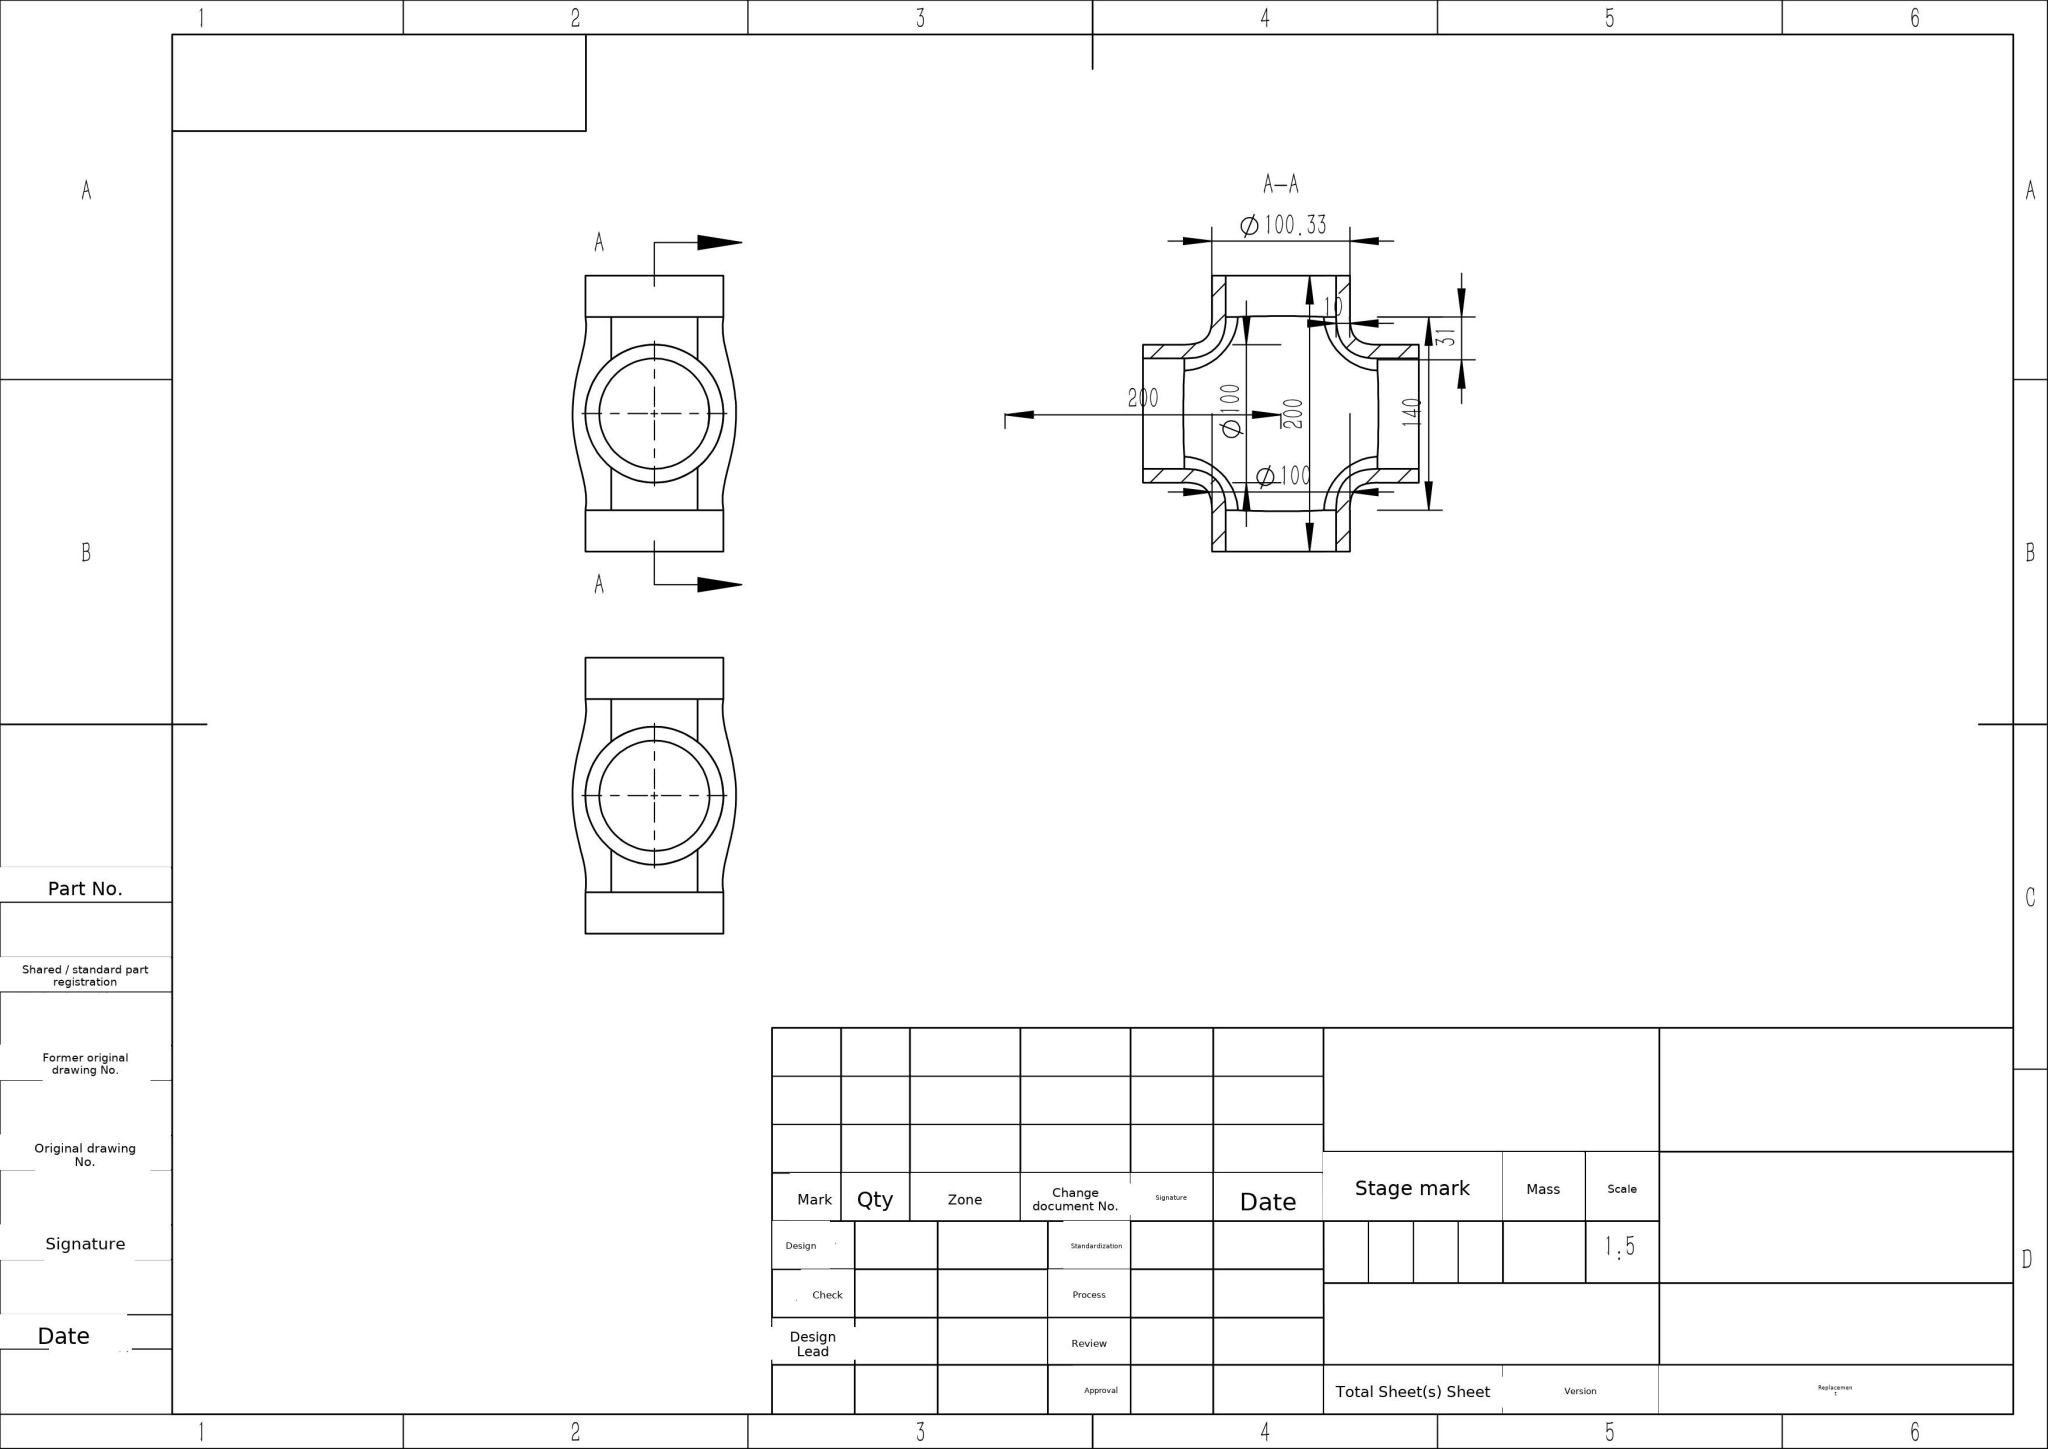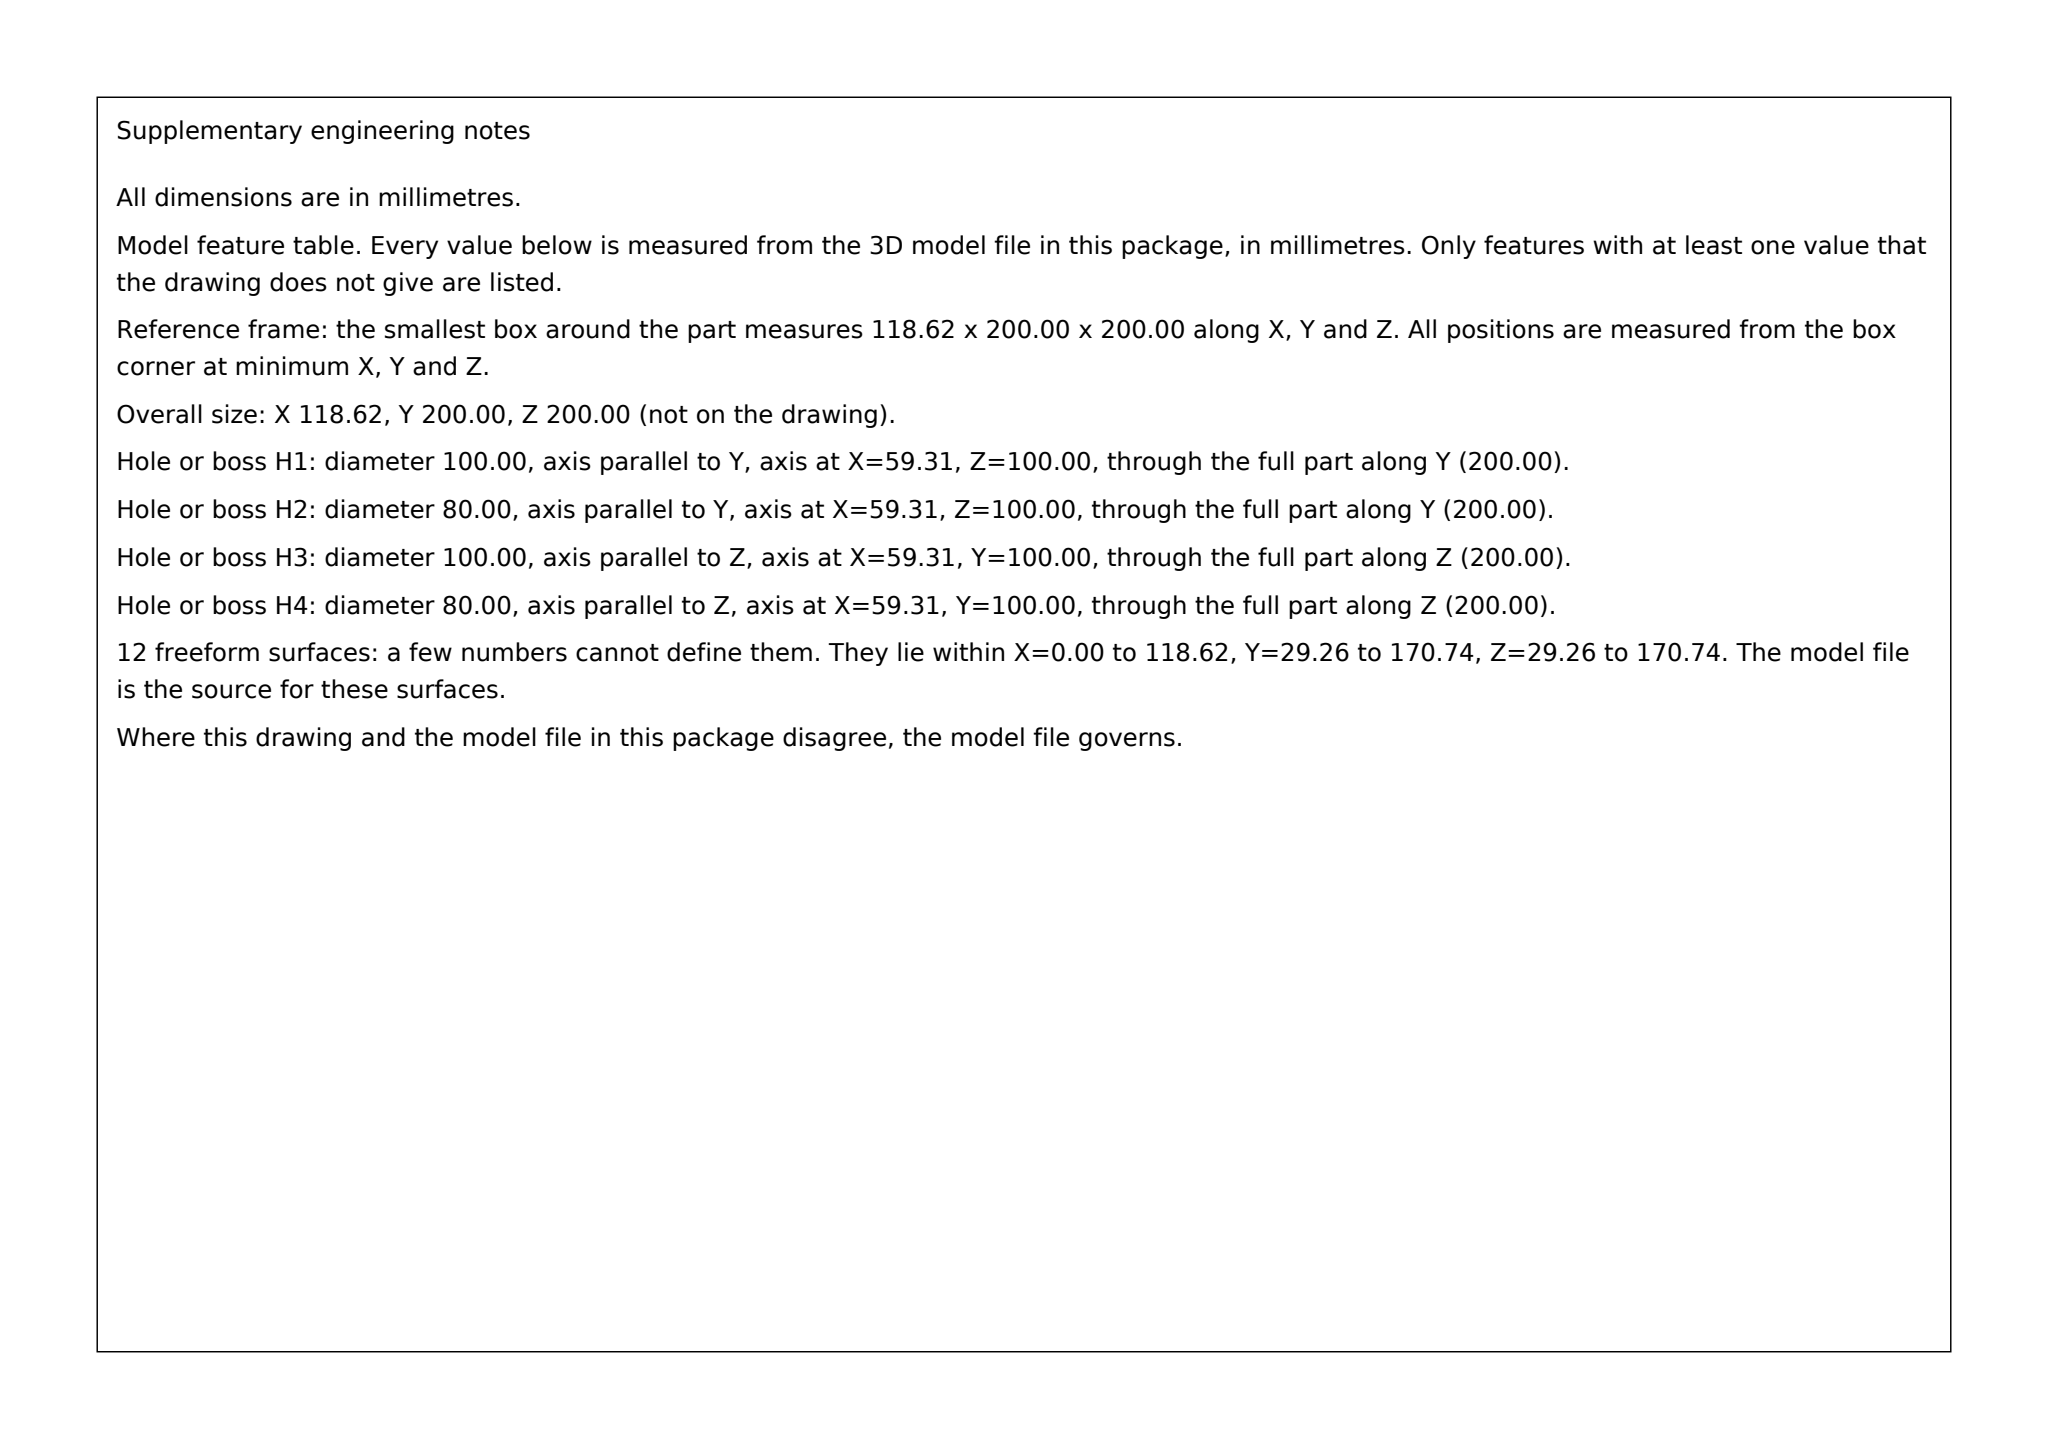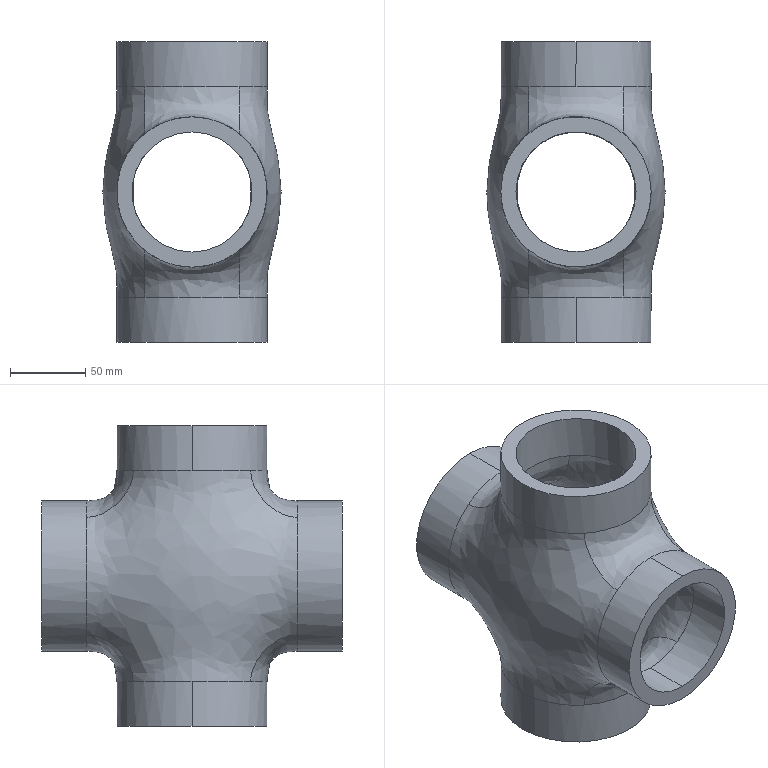Part | SolidWorks | mm | 1 solid | 32 faces | box 118.62 x 200 x 200 mm | volume 798590 mm3 | cylinder 16 | spline 12 | plane 4 | commonest cylinder face diameters 80 x8 100 x8